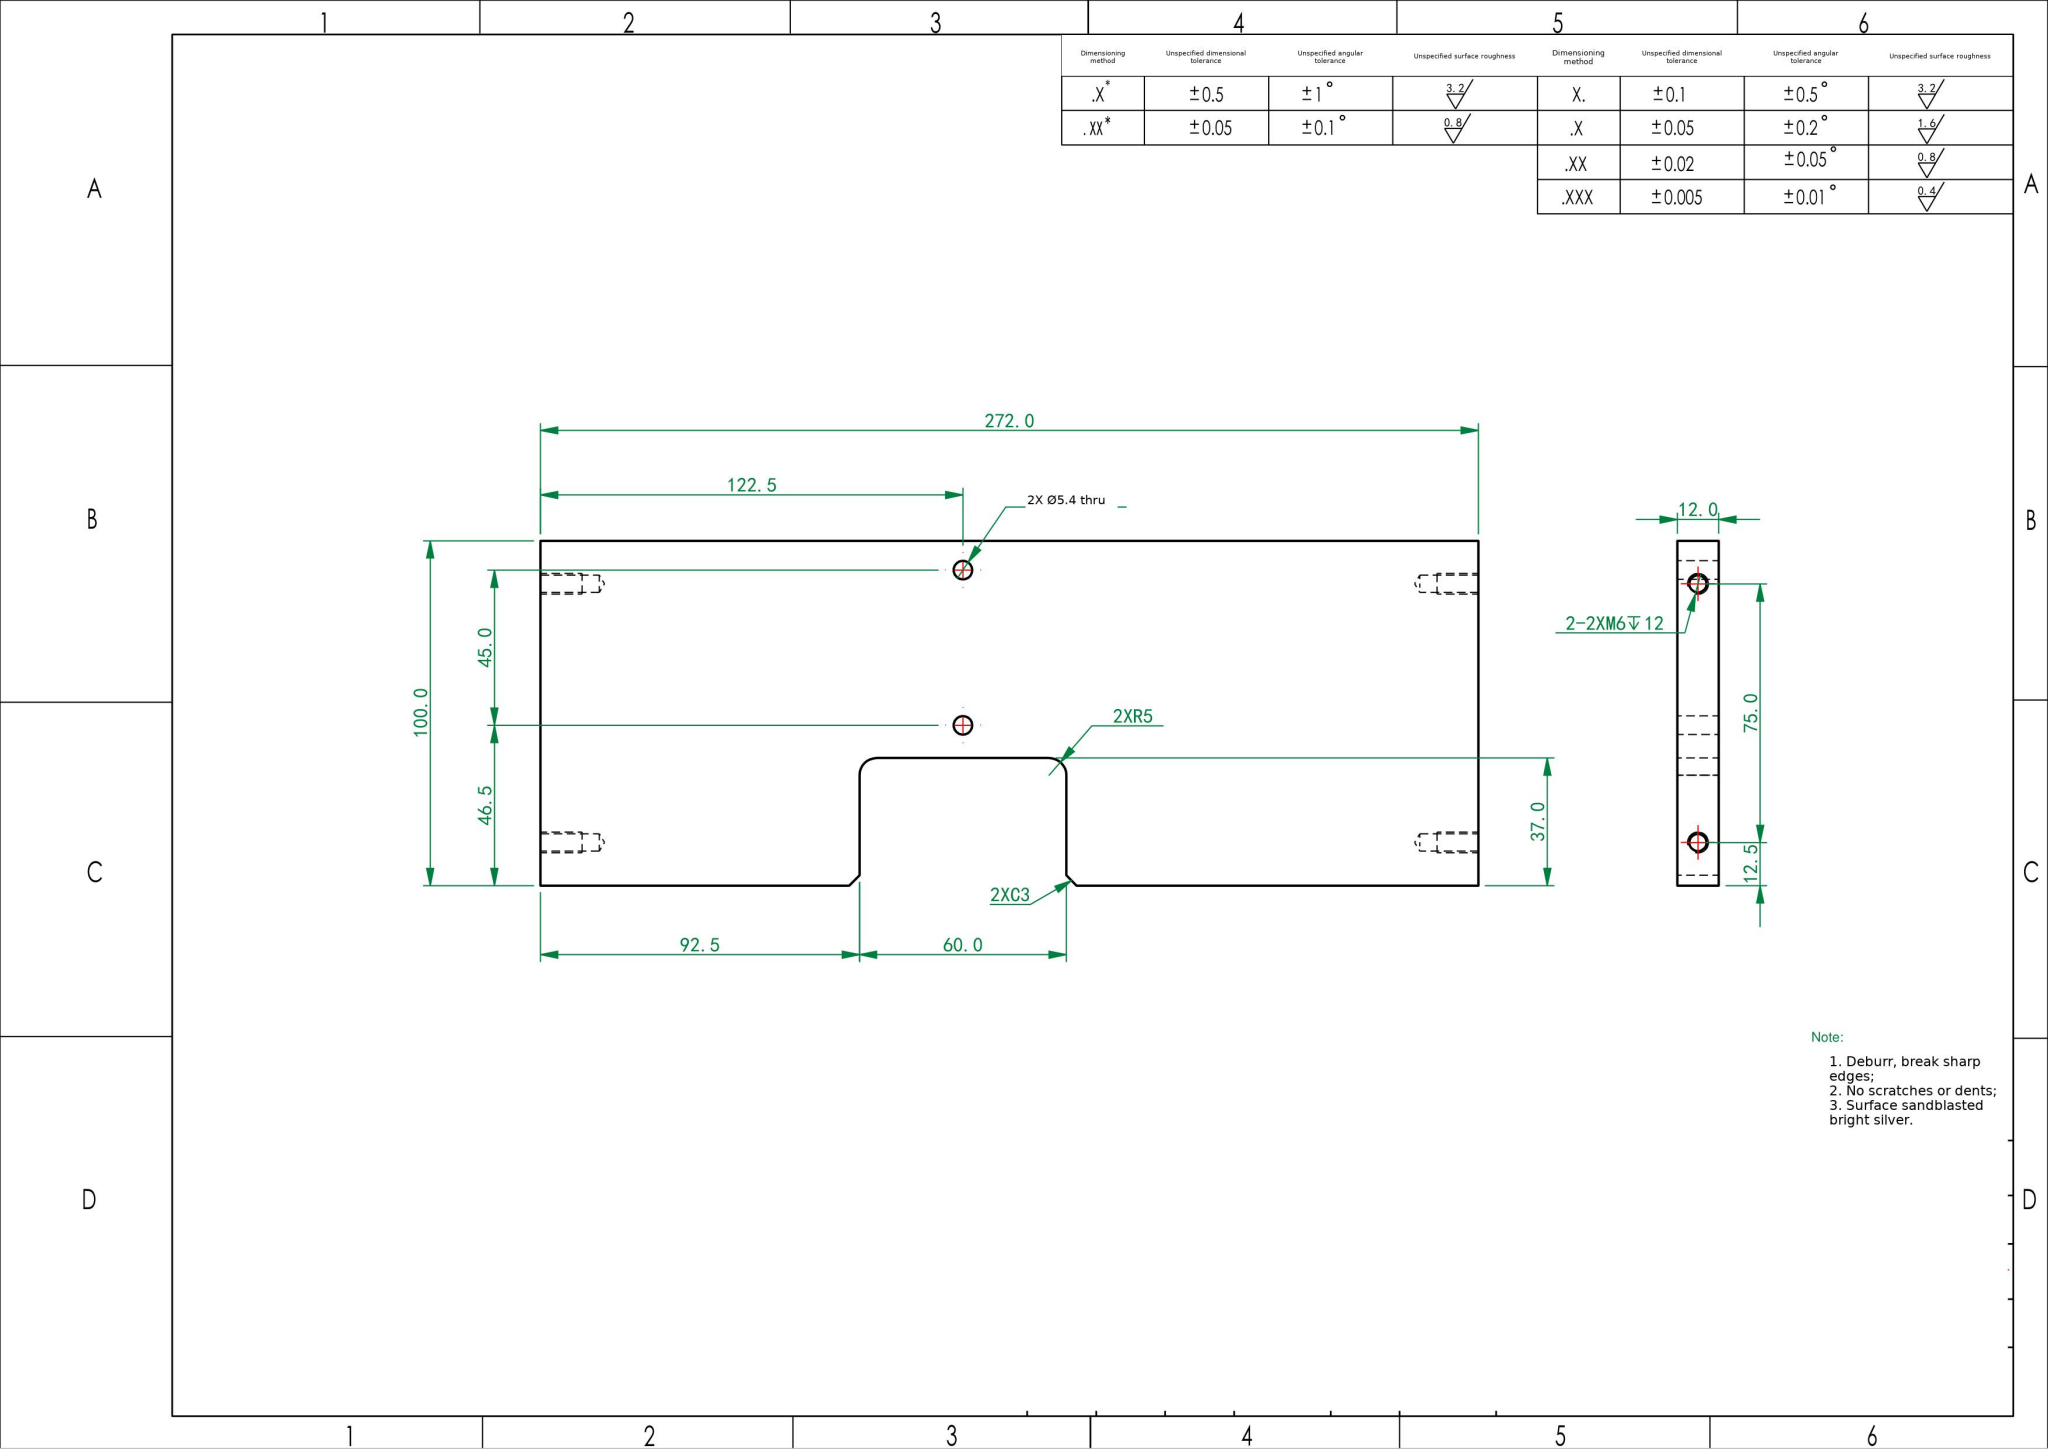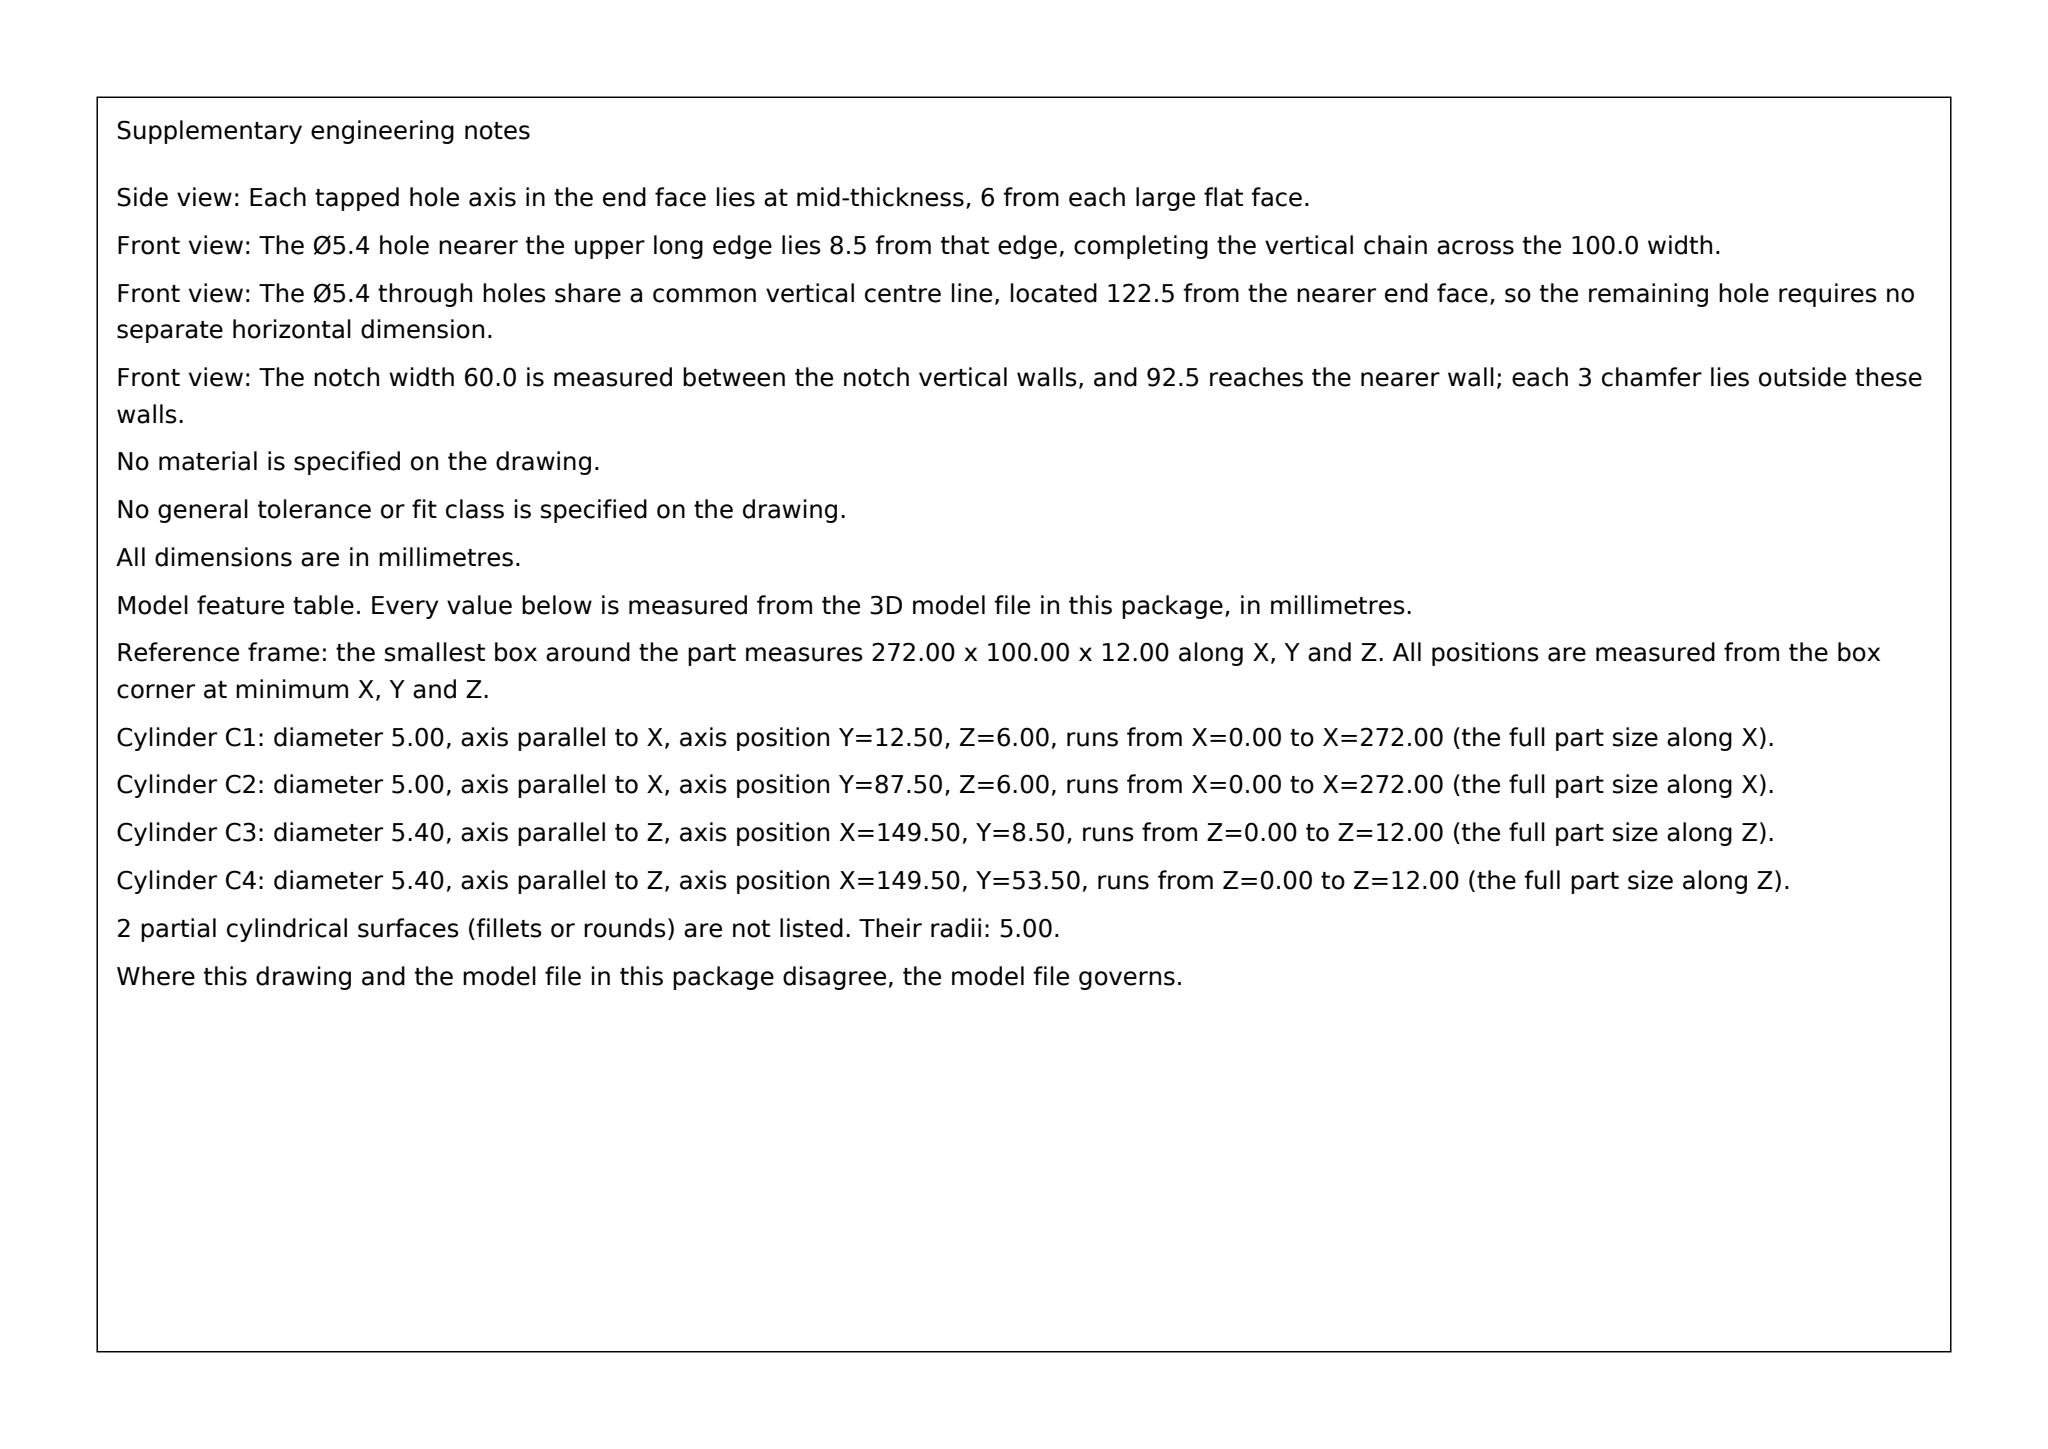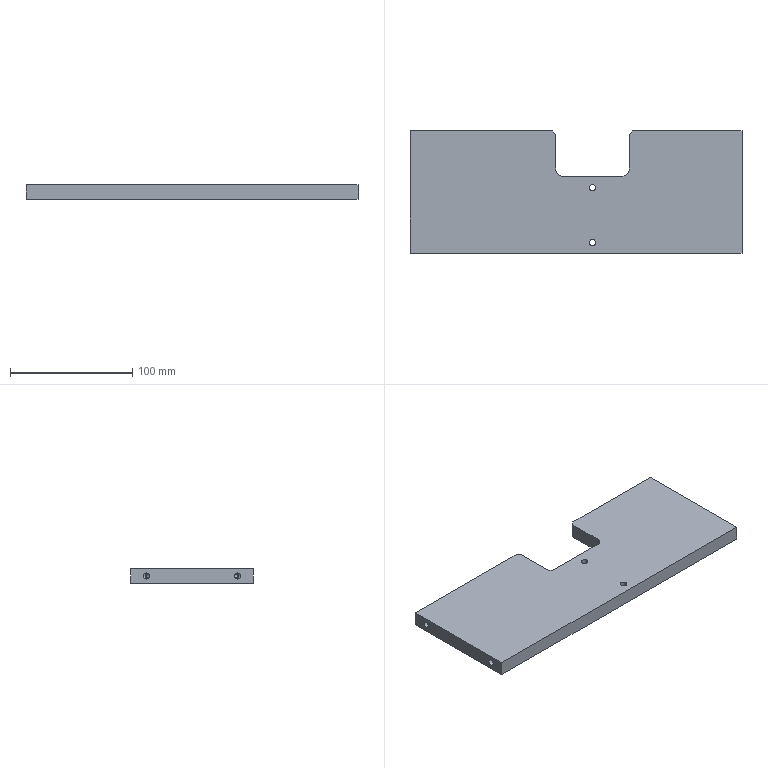Part | SolidWorks | mm | 1 solid | 34 faces | box 272 x 100 x 12 mm | volume 297857 mm3 | cylinder 14 | plane 12 | cone 8 | commonest cylinder face diameters 5 x8 5.4 x4 10 x2
Drawing notes:
SIDE VIEW: TAPPED HOLE AXES AT 6.0 FROM FACE, CL OF 12 THK | from the solid: Ø5.0 x-axis holes at z=6.0 in 12.0 thick plate (bbox z=12.0)
4X M6 DP 12 (2 EA END), TAP DRILL Ø5 DP 17 | from the solid: Ø5.0 cyls along x, len 17.0, at y=12.5 and y=87.5, both ends (4 holes)
2X Ø5.4 THRU 12 THK, UNTAPPED; M6 TAPS ARE IN ENDS ONLY | from the solid: Ø5.4 z-axis cyls at x=149.5, y=8.5 & 53.5, length 12.0 = full thk
build123d program:
from build123d import *

# Parameters (mm, degrees)
SKETCH1_W                  = 272
SKETCH1_H                  = 100
BOSS_EXTRUDE1_DEPTH        = 6
M6_TAPPED_HOLE1_AT_2_COUNT = 2
M6_TAPPED_HOLE1_AT_2_PITCH = 75
F_5_4_5_4_DIAMETER_HOLE2_D = 5.4
SKETCH10_W                 = 60
SKETCH10_H                 = 74
CUT_EXTRUDE2_DEPTH         = 55
FILLET1_R                  = 5
CHAMFER1_SIZE              = 3


with BuildPart() as part:
    # Sketch1 → Boss-Extrude1 (new, symmetric)
    with BuildSketch(Plane.XY):
        Rectangle(SKETCH1_W, SKETCH1_H)
    extrude(amount=BOSS_EXTRUDE1_DEPTH, both=True)

    # Sketch3 → M6 Tapped Hole1 (revolve, cut)
    with BuildSketch(Plane(origin=(136, 37.5, 0), x_dir=(0, 0, -1), z_dir=(0, 1, 0))):
        Polygon((0, 0), (0, 18.502), (2.5, 17), (2.5, 0), align=None)
    m6_tapped_hole1 = revolve(axis=Axis((142.35, 37.5, 0), (-1, 0, 0)), mode=Mode.SUBTRACT)

    # M6 Tapped Hole1 at 2: M6 Tapped Hole1 ×2
    with Locations(*[(0, -i * M6_TAPPED_HOLE1_AT_2_PITCH, 0) for i in range(1, M6_TAPPED_HOLE1_AT_2_COUNT)]):
        add(m6_tapped_hole1, mode=Mode.SUBTRACT)

    # Mirror1: M6 Tapped Hole1 across plane
    add(m6_tapped_hole1.mirror(Plane(origin=(0, 0, 0), x_dir=(0, 0, 1), z_dir=(1, 0, 0))), mode=Mode.SUBTRACT)

    # Mirror1 copy 1 sketch → Mirror1 copy 1 (revolve, cut)
    with BuildSketch(Plane(origin=(-136, -37.5, 0), x_dir=(0, 0, -1), z_dir=(0, 1, 0))):
        Polygon((0, 0), (0, -18.502), (2.5, -17), (2.5, 0), align=None)
    revolve(axis=Axis((-142.35, -37.5, 0), (-1, 0, 0)), mode=Mode.SUBTRACT)

    # 5.4 _5.4_ Diameter Hole2 (through all)
    with Locations(Plane(origin=(13.5, 3.5, -6), x_dir=(-1, 0, 0), z_dir=(0, 0, -1))):
        with Locations((0, 0), (0, -45)):
            Hole(F_5_4_5_4_DIAMETER_HOLE2_D / 2)

    # Sketch10 → Cut-Extrude2 (cut)
    with BuildSketch(Plane(origin=(0, 0, -6), x_dir=(-1, 0, 0), z_dir=(0, 0, -1))):
        with Locations((-13.5, 50)):
            Rectangle(SKETCH10_W, SKETCH10_H)
    extrude(amount=-CUT_EXTRUDE2_DEPTH, mode=Mode.SUBTRACT)

    # Fillet1
    fillet1_edges = [part.edges().sort_by_distance(p)[0] for p in [
        (43.5, 13, 0),
        (-16.5, 13, 0),
    ]]
    fillet(fillet1_edges, radius=FILLET1_R)

    # Chamfer1
    chamfer1_edges = [part.edges().sort_by_distance(p)[0] for p in [
        (-16.5, 50, 0),
        (43.5, 50, 0),
    ]]
    chamfer(chamfer1_edges, length=CHAMFER1_SIZE)


solid = part.part